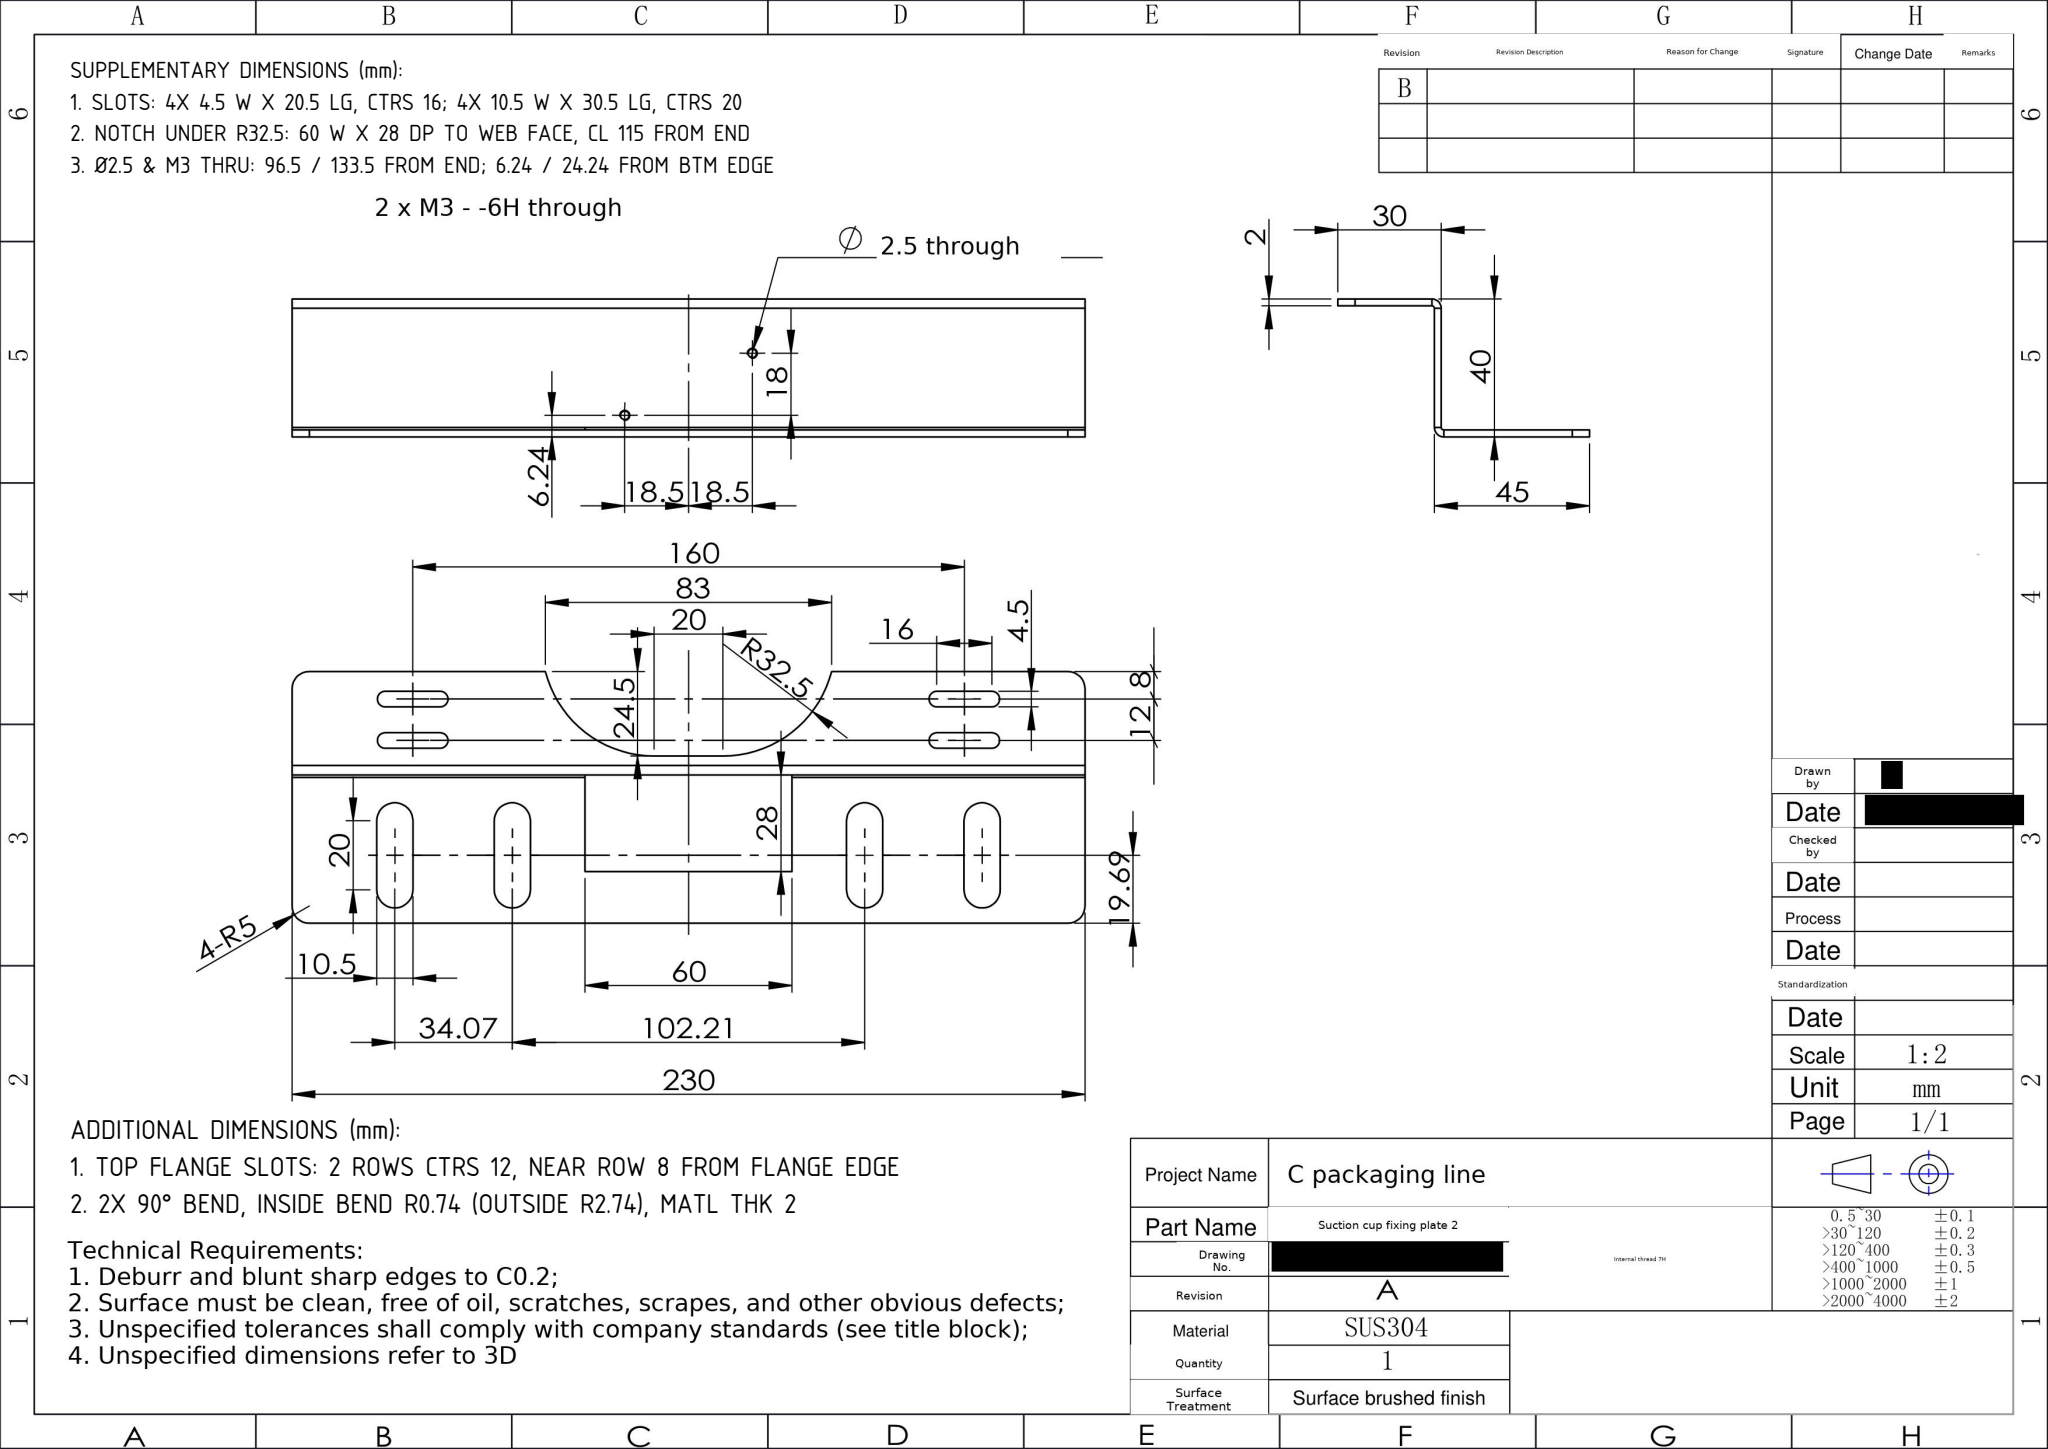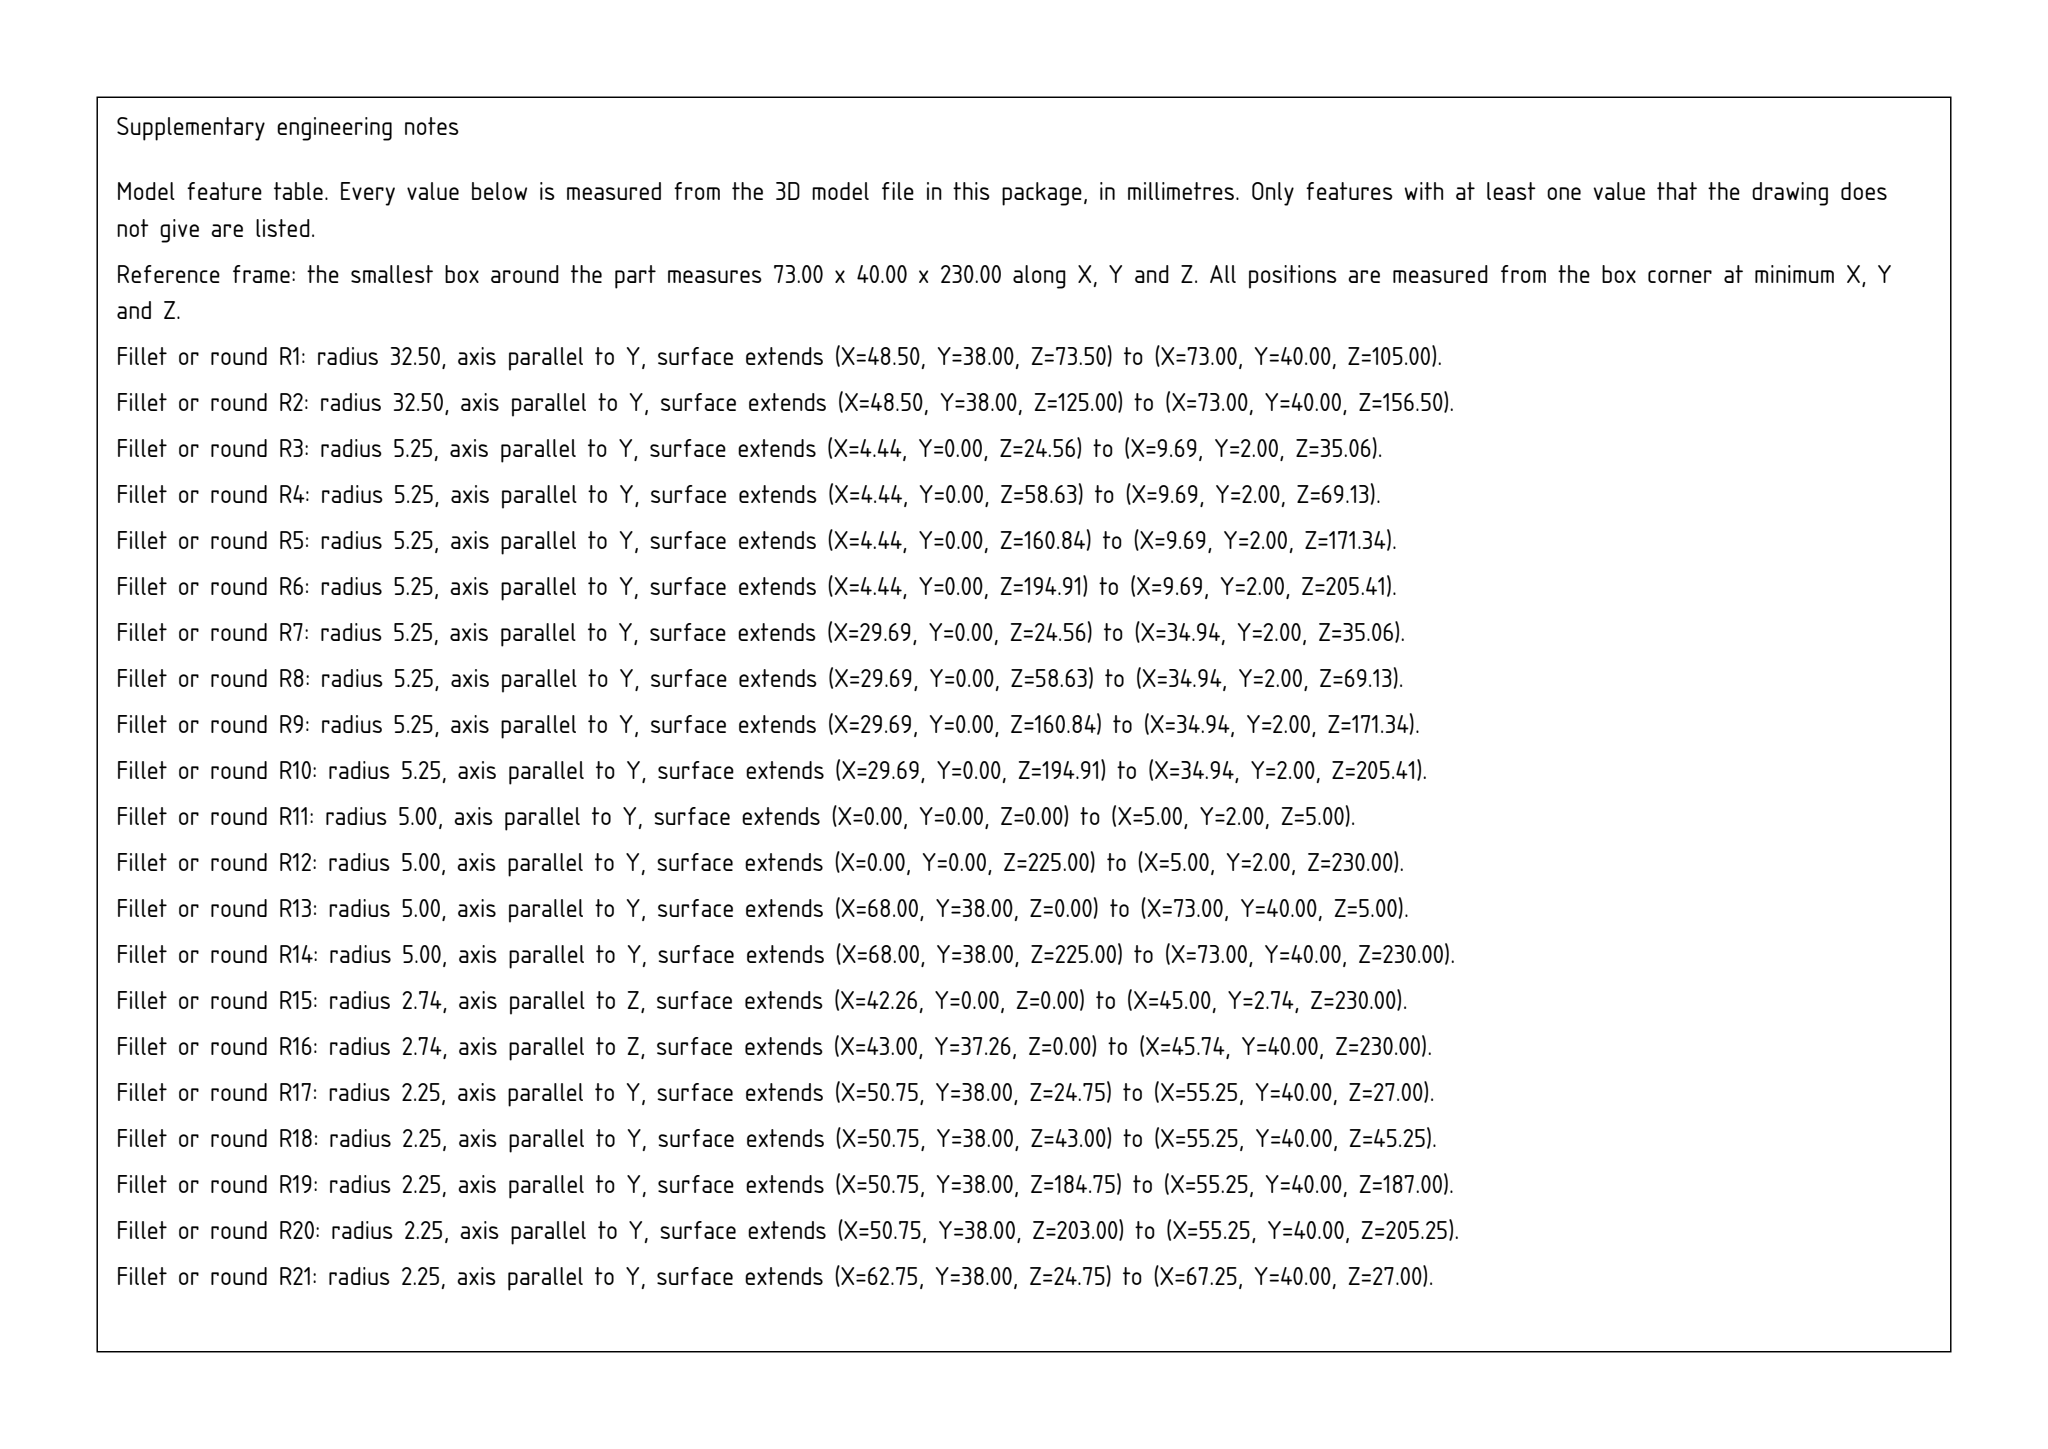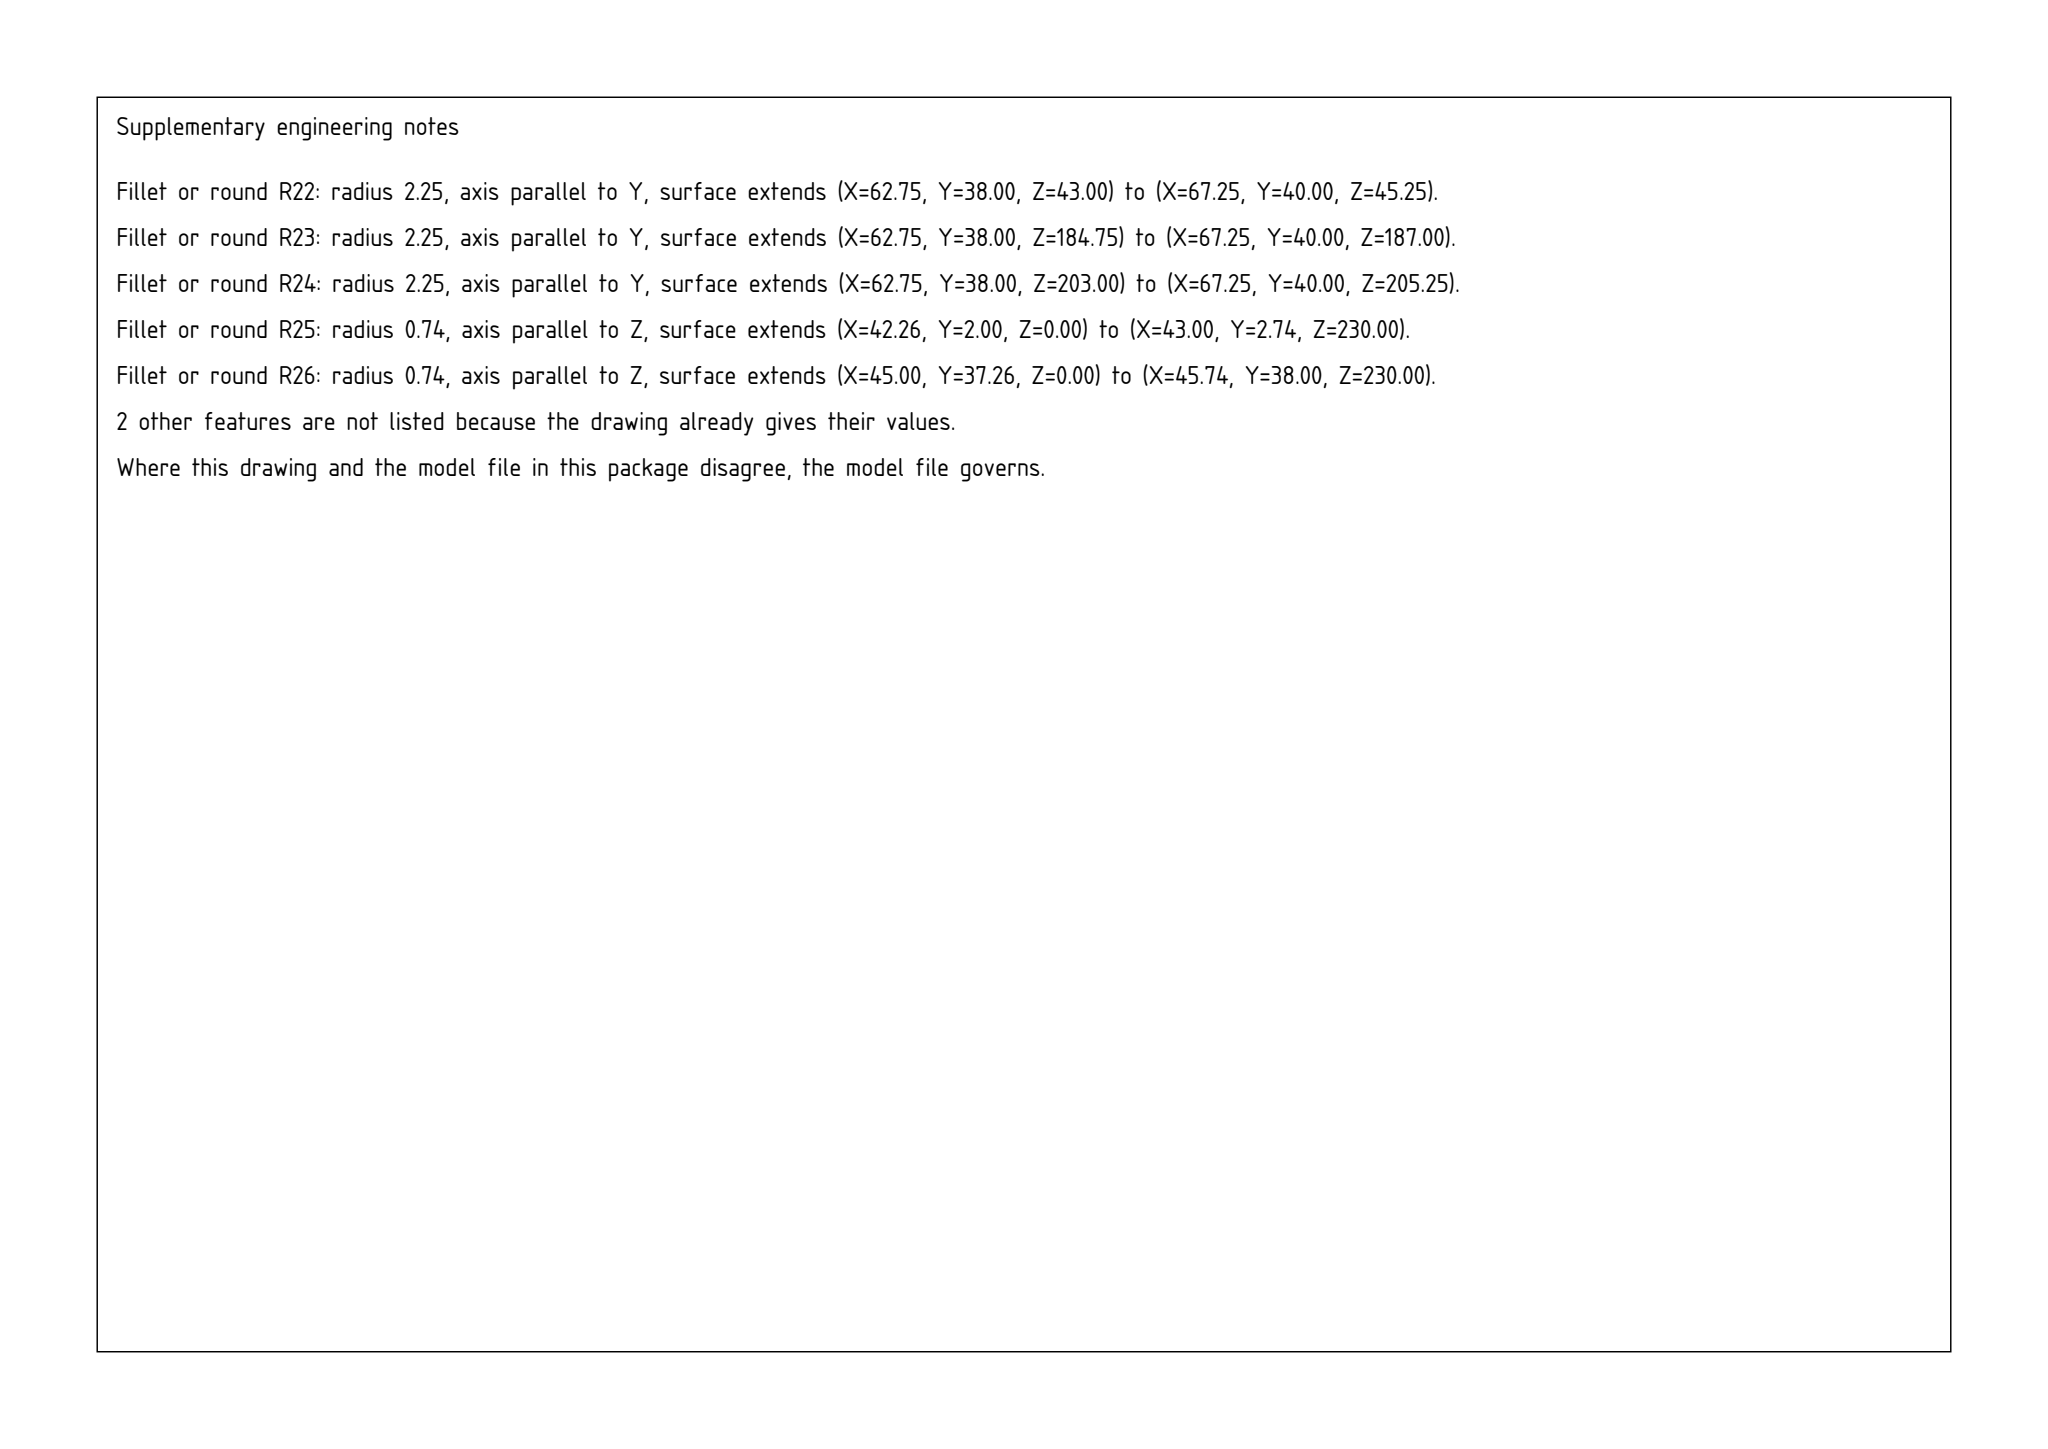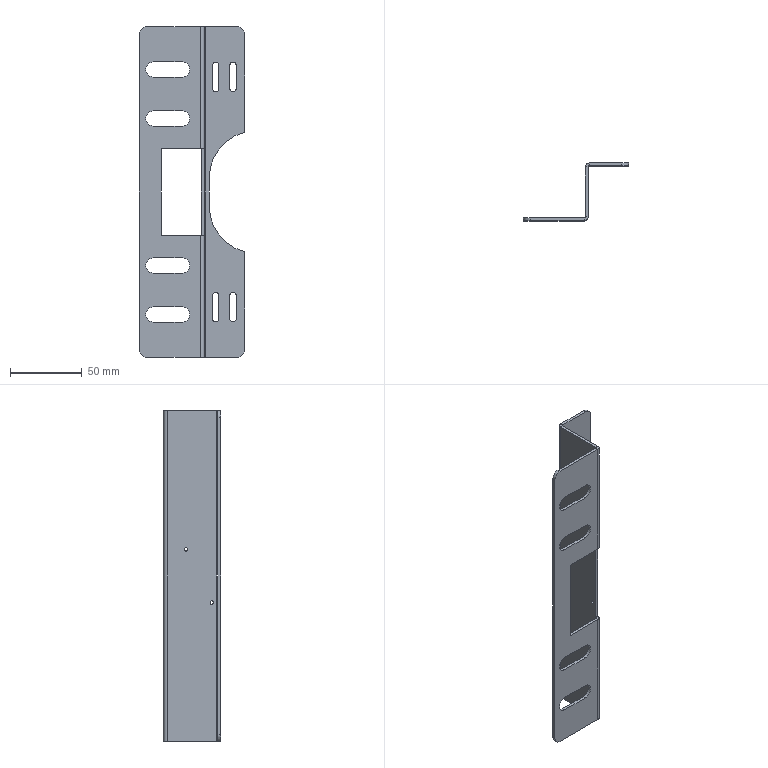Part | SolidWorks | mm | 1 solid | 76 faces | box 73 x 40 x 230 mm | volume 40368 mm3 | plane 40 | cylinder 36 | commonest cylinder face diameters 4.5 x12 10.5 x8 2.5 x4 10 x4 5.473 x3 1.473 x3 65 x2